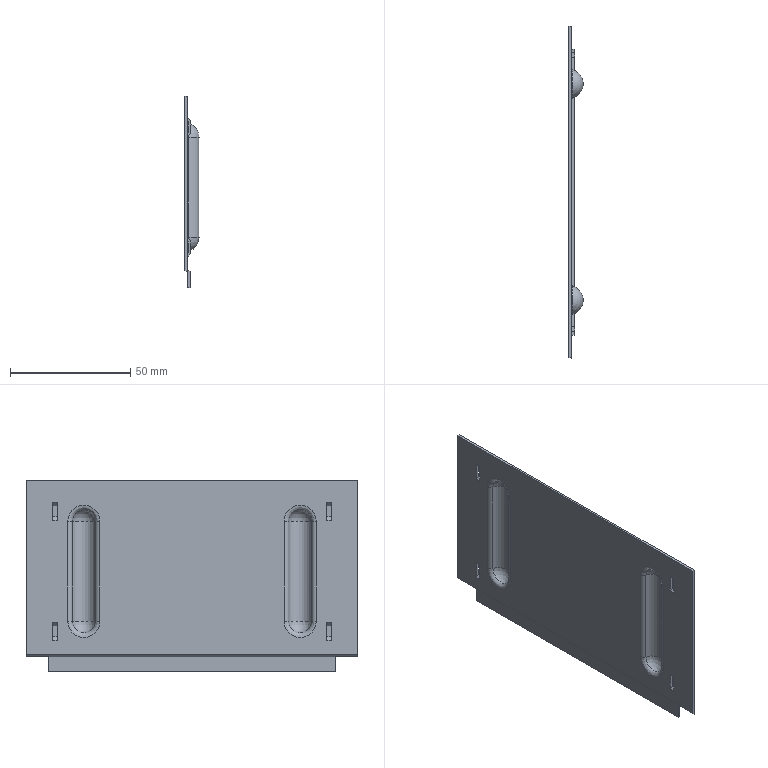Component | NX | SIDE_PANEL | 1 solid | 80 faces | volume 11464 mm3 | plane 52 | cylinder 12 | sphere 8 | torus 8 | commonest cylinder face diameters 4 x4 2 x4 10 x2 12 x2